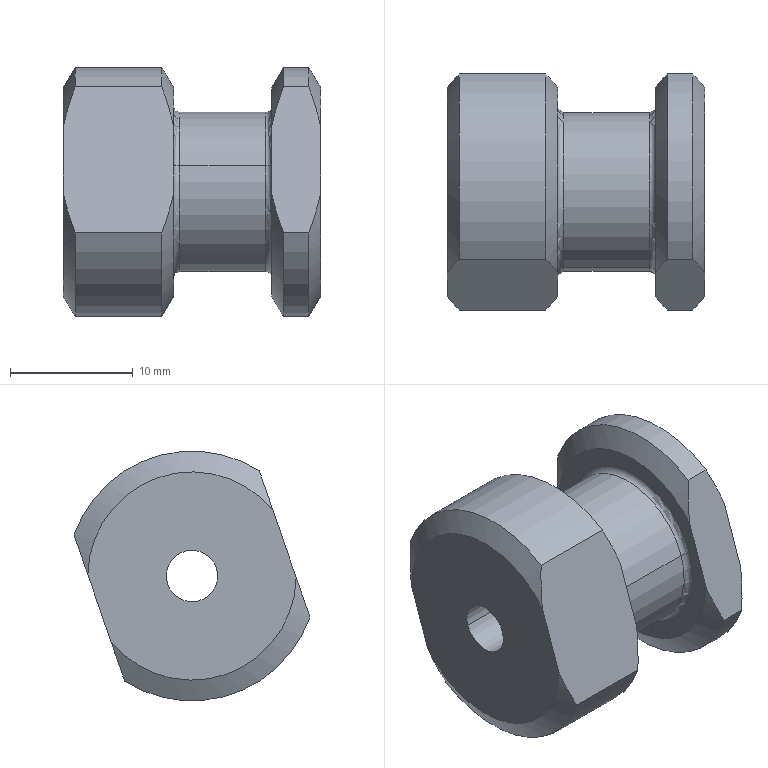Component | SolidWorks | 06-1111-1 | 1 solid | 28 faces | box 21 x 19.26 x 20.38 mm | volume 4401 mm3 | cylinder 8 | cone 8 | plane 8 | torus 4 | commonest cylinder face diameters 20.384 x4 4.2 x2 13 x2
build123d program:
from build123d import *

# Parameters (mm, degrees)
SKETCH2_OUTSIDE_W   = 29.518
SKETCH2_OUTSIDE_H   = 29.518
SKETCH2_OUTSIDE_W_2 = 16
SKETCH2_OUTSIDE_H_2 = 25
EXTRUDE1_DEPTH      = 22
M5_TAPPED_HOLE1_D   = 4.2


with BuildPart() as part:
    # Sketch1 → Revolve1 (revolve)
    with BuildSketch(Plane.XY, mode=Mode.PRIVATE) as revolve1_sk:
        with BuildLine():
            Line((0, 0), (0, 8.5))
            Line((0, 8.5), (0.9769, 10.192))
            Line((0.9769, 10.192), (3.023, 10.192))
            Line((3.023, 10.192), (4, 8.5))
            Line((4, 8.5), (4, 7))
            ThreePointArc((4, 7), (4.146, 6.646), (4.5, 6.5))
            Line((4.5, 6.5), (11.5, 6.5))
            ThreePointArc((11.5, 6.5), (11.854, 6.646), (12, 7))
            Line((12, 7), (12, 8.5))
            Line((12, 8.5), (12.977, 10.192))
            Line((12.977, 10.192), (20.023, 10.192))
            Line((20.023, 10.192), (21, 8.5))
            Line((21, 8.5), (21, 0))
            Line((21, 0), (0, 0))
        make_face()
    revolve(revolve1_sk.sketch.rotate(Axis((21, 0, 0), (-1, 0, 0)), 270), axis=Axis((21, 0, 0), (-1, 0, 0)))

    # Sketch2 outside → Extrude1 (cut)
    with BuildSketch(Plane(origin=(0, 0, 0), x_dir=(0, 0, -1), z_dir=(1, 0, 0))):
        Rectangle(SKETCH2_OUTSIDE_W, SKETCH2_OUTSIDE_H)
        Rectangle(SKETCH2_OUTSIDE_W_2, SKETCH2_OUTSIDE_H_2, mode=Mode.SUBTRACT)
    extrude(amount=EXTRUDE1_DEPTH, mode=Mode.SUBTRACT)

    # M5 Tapped Hole1 (through all)
    with Locations(Plane.ZY):
        with Locations((0, 0)):
            Hole(M5_TAPPED_HOLE1_D / 2)


solid = part.part

# Placed as in the assembly
solid = solid.moved(Location((-65, 24, -26), (-109.129, 0, 180)))
STEP:
#1=CARTESIAN_POINT('',(-3.386,0.8668,-0.9965));
#2=VERTEX_POINT('',#1);
#3=CARTESIAN_POINT('',(-3.386,1.023,-1.051));
#4=VERTEX_POINT('',#3);
#5=CARTESIAN_POINT('',(-3.386,0.9449,-1.024));
#6=DIRECTION('',(1.,0.,-0.));
#7=DIRECTION('',(0.,0.9448,-0.3277));
#8=AXIS2_PLACEMENT_3D('',#5,#6,#7);
#9=CIRCLE('',#8,0.08268);
#10=EDGE_CURVE('',#2,#4,#9,.T.);
#11=ORIENTED_EDGE('',*,*,#10,.F.);
#12=CARTESIAN_POINT('',(-2.559,0.8668,-0.9965));
#13=VERTEX_POINT('',#12);
#14=CARTESIAN_POINT('',(-2.559,0.8668,-0.9965));
#15=DIRECTION('',(1.,0.,-0.));
#16=VECTOR('',#15,39.37);
#17=LINE('',#14,#16);
#18=EDGE_CURVE('',#2,#13,#17,.T.);
#19=ORIENTED_EDGE('',*,*,#18,.T.);
#20=CARTESIAN_POINT('',(-2.559,1.023,-1.051));
#21=VERTEX_POINT('',#20);
#22=CARTESIAN_POINT('',(-2.559,0.9449,-1.024));
#23=DIRECTION('',(1.,0.,-0.));
#24=DIRECTION('',(0.,0.9448,-0.3277));
#25=AXIS2_PLACEMENT_3D('',#22,#23,#24);
#26=CIRCLE('',#25,0.08268);
#27=EDGE_CURVE('',#13,#21,#26,.T.);
#28=ORIENTED_EDGE('',*,*,#27,.T.);
#29=CARTESIAN_POINT('',(-2.559,1.023,-1.051));
#30=DIRECTION('',(1.,0.,-0.));
#31=VECTOR('',#30,39.37);
#32=LINE('',#29,#31);
#33=EDGE_CURVE('',#4,#21,#32,.T.);
#34=ORIENTED_EDGE('',*,*,#33,.F.);
#35=EDGE_LOOP('',(#11,#19,#28,#34));
#36=FACE_OUTER_BOUND('',#35,.T.);
#37=CARTESIAN_POINT('',(-2.559,0.9449,-1.024));
#38=DIRECTION('',(1.,0.,-0.));
#39=DIRECTION('',(0.,0.9448,-0.3277));
#40=AXIS2_PLACEMENT_3D('',#37,#38,#39);
#41=CYLINDRICAL_SURFACE('',#40,0.08268);
#42=ADVANCED_FACE('',(#36),#41,.F.);
#43=CARTESIAN_POINT('',(-2.717,0.6845,-0.9333));
#44=VERTEX_POINT('',#43);
#45=CARTESIAN_POINT('',(-2.717,1.205,-1.114));
#46=VERTEX_POINT('',#45);
#47=CARTESIAN_POINT('',(-2.717,0.9449,-1.024));
#48=DIRECTION('',(1.,0.,-0.));
#49=DIRECTION('',(0.,0.9448,-0.3277));
#50=AXIS2_PLACEMENT_3D('',#47,#48,#49);
#51=CIRCLE('',#50,0.2756);
#52=EDGE_CURVE('',#44,#46,#51,.T.);
#53=ORIENTED_EDGE('',*,*,#52,.F.);
#54=CARTESIAN_POINT('',(-2.736,0.7031,-0.9398));
#55=VERTEX_POINT('',#54);
#56=CARTESIAN_POINT('',(-2.736,0.6845,-0.9333));
#57=DIRECTION('',(0.,0.3277,0.9448));
#58=DIRECTION('',(0.,-0.9448,0.3277));
#59=AXIS2_PLACEMENT_3D('',#56,#57,#58);
#60=CIRCLE('',#59,0.01969);
#61=EDGE_CURVE('',#44,#55,#60,.T.);
#62=ORIENTED_EDGE('',*,*,#61,.T.);
#63=CARTESIAN_POINT('',(-2.736,1.187,-1.107));
#64=VERTEX_POINT('',#63);
#65=CARTESIAN_POINT('',(-2.736,0.9449,-1.024));
#66=DIRECTION('',(1.,0.,-0.));
#67=DIRECTION('',(0.,0.9448,-0.3277));
#68=AXIS2_PLACEMENT_3D('',#65,#66,#67);
#69=CIRCLE('',#68,0.2559);
#70=EDGE_CURVE('',#55,#64,#69,.T.);
#71=ORIENTED_EDGE('',*,*,#70,.T.);
#72=CARTESIAN_POINT('',(-2.736,1.205,-1.114));
#73=DIRECTION('',(-0.,-0.3277,-0.9448));
#74=DIRECTION('',(0.,0.9448,-0.3277));
#75=AXIS2_PLACEMENT_3D('',#72,#73,#74);
#76=CIRCLE('',#75,0.01969);
#77=EDGE_CURVE('',#46,#64,#76,.T.);
#78=ORIENTED_EDGE('',*,*,#77,.F.);
#79=EDGE_LOOP('',(#53,#62,#71,#78));
#80=FACE_OUTER_BOUND('',#79,.T.);
#81=CARTESIAN_POINT('',(-2.736,0.9449,-1.024));
#82=DIRECTION('',(1.,0.,-0.));
#83=DIRECTION('',(-0.,0.9448,-0.3277));
#84=AXIS2_PLACEMENT_3D('',#81,#82,#83);
#85=TOROIDAL_SURFACE('',#84,0.2756,0.01969);
#86=ADVANCED_FACE('',(#80),#85,.F.);
#87=CARTESIAN_POINT('',(-3.012,1.187,-1.107));
#88=VERTEX_POINT('',#87);
#89=CARTESIAN_POINT('',(-3.012,0.7031,-0.9398));
#90=VERTEX_POINT('',#89);
#91=CARTESIAN_POINT('',(-3.012,0.9449,-1.024));
#92=DIRECTION('',(1.,0.,-0.));
#93=DIRECTION('',(0.,0.9448,-0.3277));
#94=AXIS2_PLACEMENT_3D('',#91,#92,#93);
#95=CIRCLE('',#94,0.2559);
#96=EDGE_CURVE('',#88,#90,#95,.T.);
#97=ORIENTED_EDGE('',*,*,#96,.T.);
#98=CARTESIAN_POINT('',(-3.386,0.7031,-0.9398));
#99=DIRECTION('',(1.,0.,-0.));
#100=VECTOR('',#99,39.37);
#101=LINE('',#98,#100);
#102=EDGE_CURVE('',#90,#55,#101,.T.);
#103=ORIENTED_EDGE('',*,*,#102,.T.);
#104=CARTESIAN_POINT('',(-2.736,0.9449,-1.024));
#105=DIRECTION('',(1.,0.,-0.));
#106=DIRECTION('',(0.,0.9448,-0.3277));
#107=AXIS2_PLACEMENT_3D('',#104,#105,#106);
#108=CIRCLE('',#107,0.2559);
#109=EDGE_CURVE('',#64,#55,#108,.T.);
#110=ORIENTED_EDGE('',*,*,#109,.F.);
#111=CARTESIAN_POINT('',(-3.386,1.187,-1.107));
#112=DIRECTION('',(1.,0.,-0.));
#113=VECTOR('',#112,39.37);
#114=LINE('',#111,#113);
#115=EDGE_CURVE('',#88,#64,#114,.T.);
#116=ORIENTED_EDGE('',*,*,#115,.F.);
#117=EDGE_LOOP('',(#97,#103,#110,#116));
#118=FACE_OUTER_BOUND('',#117,.T.);
#119=CARTESIAN_POINT('',(-3.386,0.9449,-1.024));
#120=DIRECTION('',(1.,0.,-0.));
#121=DIRECTION('',(0.,0.9448,-0.3277));
#122=AXIS2_PLACEMENT_3D('',#119,#120,#121);
#123=CYLINDRICAL_SURFACE('',#122,0.2559);
#124=ADVANCED_FACE('',(#118),#123,.T.);
#125=CARTESIAN_POINT('',(-3.012,0.9449,-1.024));
#126=DIRECTION('',(1.,0.,-0.));
#127=DIRECTION('',(0.,0.9448,-0.3277));
#128=AXIS2_PLACEMENT_3D('',#125,#126,#127);
#129=CIRCLE('',#128,0.2559);
#130=EDGE_CURVE('',#90,#88,#129,.T.);
#131=ORIENTED_EDGE('',*,*,#130,.F.);
#132=CARTESIAN_POINT('',(-3.031,0.6845,-0.9333));
#133=VERTEX_POINT('',#132);
#134=CARTESIAN_POINT('',(-3.012,0.6845,-0.9333));
#135=DIRECTION('',(0.,0.3277,0.9448));
#136=DIRECTION('',(0.,-0.9448,0.3277));
#137=AXIS2_PLACEMENT_3D('',#134,#135,#136);
#138=CIRCLE('',#137,0.01969);
#139=EDGE_CURVE('',#90,#133,#138,.T.);
#140=ORIENTED_EDGE('',*,*,#139,.T.);
#141=CARTESIAN_POINT('',(-3.031,1.205,-1.114));
#142=VERTEX_POINT('',#141);
#143=CARTESIAN_POINT('',(-3.031,0.9449,-1.024));
#144=DIRECTION('',(1.,0.,-0.));
#145=DIRECTION('',(0.,0.9448,-0.3277));
#146=AXIS2_PLACEMENT_3D('',#143,#144,#145);
#147=CIRCLE('',#146,0.2756);
#148=EDGE_CURVE('',#133,#142,#147,.T.);
#149=ORIENTED_EDGE('',*,*,#148,.T.);
#150=CARTESIAN_POINT('',(-3.012,1.205,-1.114));
#151=DIRECTION('',(-0.,-0.3277,-0.9448));
#152=DIRECTION('',(0.,0.9448,-0.3277));
#153=AXIS2_PLACEMENT_3D('',#150,#151,#152);
#154=CIRCLE('',#153,0.01969);
#155=EDGE_CURVE('',#88,#142,#154,.T.);
#156=ORIENTED_EDGE('',*,*,#155,.F.);
#157=EDGE_LOOP('',(#131,#140,#149,#156));
#158=FACE_OUTER_BOUND('',#157,.T.);
#159=CARTESIAN_POINT('',(-3.012,0.9449,-1.024));
#160=DIRECTION('',(1.,0.,-0.));
#161=DIRECTION('',(-0.,0.9448,-0.3277));
#162=AXIS2_PLACEMENT_3D('',#159,#160,#161);
#163=TOROIDAL_SURFACE('',#162,0.2756,0.01969);
#164=ADVANCED_FACE('',(#158),#163,.F.);
#165=CARTESIAN_POINT('',(-3.347,1.324,-0.8919));
#166=VERTEX_POINT('',#165);
#167=CARTESIAN_POINT('',(-3.347,0.7288,-0.6855));
#168=VERTEX_POINT('',#167);
#169=CARTESIAN_POINT('',(-3.347,0.9449,-1.024));
#170=DIRECTION('',(1.,0.,-0.));
#171=DIRECTION('',(0.,0.9448,-0.3277));
#172=AXIS2_PLACEMENT_3D('',#169,#170,#171);
#173=CIRCLE('',#172,0.4013);
#174=EDGE_CURVE('',#166,#168,#173,.T.);
#175=ORIENTED_EDGE('',*,*,#174,.F.);
#176=CARTESIAN_POINT('',(-3.386,1.28,-1.02));
#177=VERTEX_POINT('',#176);
#178=CARTESIAN_POINT('',(-3.347,1.324,-0.8919));
#179=CARTESIAN_POINT('',(-3.355,1.317,-0.9128));
#180=CARTESIAN_POINT('',(-3.363,1.309,-0.9338));
#181=CARTESIAN_POINT('',(-3.376,1.295,-0.9765));
#182=CARTESIAN_POINT('',(-3.381,1.287,-0.9981));
#183=CARTESIAN_POINT('',(-3.386,1.28,-1.02));
#184=B_SPLINE_CURVE_WITH_KNOTS('',3,(#178,#179,#180,#181,#182,#183),.UNSPECIFIED.,.F.,.F.,(4,2,4),(0.01795,0.01974,0.02153),.UNSPECIFIED.);
#185=EDGE_CURVE('',#166,#177,#184,.T.);
#186=ORIENTED_EDGE('',*,*,#185,.T.);
#187=CARTESIAN_POINT('',(-3.386,0.6844,-0.8136));
#188=VERTEX_POINT('',#187);
#189=CARTESIAN_POINT('',(-3.386,0.9449,-1.024));
#190=DIRECTION('',(1.,0.,-0.));
#191=DIRECTION('',(0.,0.9448,-0.3277));
#192=AXIS2_PLACEMENT_3D('',#189,#190,#191);
#193=CIRCLE('',#192,0.3346);
#194=EDGE_CURVE('',#177,#188,#193,.T.);
#195=ORIENTED_EDGE('',*,*,#194,.T.);
#196=CARTESIAN_POINT('',(-3.386,0.6844,-0.8136));
#197=CARTESIAN_POINT('',(-3.377,0.6996,-0.7696));
#198=CARTESIAN_POINT('',(-3.363,0.7143,-0.7272));
#199=CARTESIAN_POINT('',(-3.347,0.7288,-0.6855));
#200=B_SPLINE_CURVE_WITH_KNOTS('',3,(#196,#197,#198,#199),.UNSPECIFIED.,.F.,.F.,(4,4),(0.02733,0.03094),.UNSPECIFIED.);
#201=EDGE_CURVE('',#188,#168,#200,.T.);
#202=ORIENTED_EDGE('',*,*,#201,.T.);
#203=EDGE_LOOP('',(#175,#186,#195,#202));
#204=FACE_OUTER_BOUND('',#203,.T.);
#205=CARTESIAN_POINT('',(-3.386,0.9449,-1.024));
#206=DIRECTION('',(1.,0.,-0.));
#207=DIRECTION('',(0.,0.9448,-0.3277));
#208=AXIS2_PLACEMENT_3D('',#205,#206,#207);
#209=CONICAL_SURFACE('',#208,0.3346,1.047);
#210=ADVANCED_FACE('',(#204),#209,.T.);
#211=CARTESIAN_POINT('',(-3.347,0.5658,-1.155));
#212=VERTEX_POINT('',#211);
#213=CARTESIAN_POINT('',(-3.347,1.161,-1.362));
#214=VERTEX_POINT('',#213);
#215=CARTESIAN_POINT('',(-3.347,0.9449,-1.024));
#216=DIRECTION('',(1.,0.,-0.));
#217=DIRECTION('',(0.,0.9448,-0.3277));
#218=AXIS2_PLACEMENT_3D('',#215,#216,#217);
#219=CIRCLE('',#218,0.4013);
#220=EDGE_CURVE('',#212,#214,#219,.T.);
#221=ORIENTED_EDGE('',*,*,#220,.T.);
#222=CARTESIAN_POINT('',(-3.07,1.161,-1.362));
#223=VERTEX_POINT('',#222);
#224=CARTESIAN_POINT('',(-3.386,1.161,-1.362));
#225=DIRECTION('',(1.,0.,-0.));
#226=VECTOR('',#225,39.37);
#227=LINE('',#224,#226);
#228=EDGE_CURVE('',#214,#223,#227,.T.);
#229=ORIENTED_EDGE('',*,*,#228,.T.);
#230=CARTESIAN_POINT('',(-3.07,0.5658,-1.155));
#231=VERTEX_POINT('',#230);
#232=CARTESIAN_POINT('',(-3.07,0.9449,-1.024));
#233=DIRECTION('',(1.,0.,-0.));
#234=DIRECTION('',(0.,0.9448,-0.3277));
#235=AXIS2_PLACEMENT_3D('',#232,#233,#234);
#236=CIRCLE('',#235,0.4013);
#237=EDGE_CURVE('',#231,#223,#236,.T.);
#238=ORIENTED_EDGE('',*,*,#237,.F.);
#239=CARTESIAN_POINT('',(-3.386,0.5658,-1.155));
#240=DIRECTION('',(-1.,-0.,0.));
#241=VECTOR('',#240,39.37);
#242=LINE('',#239,#241);
#243=EDGE_CURVE('',#231,#212,#242,.T.);
#244=ORIENTED_EDGE('',*,*,#243,.T.);
#245=EDGE_LOOP('',(#221,#229,#238,#244));
#246=FACE_OUTER_BOUND('',#245,.T.);
#247=CARTESIAN_POINT('',(-3.386,0.9449,-1.024));
#248=DIRECTION('',(1.,0.,-0.));
#249=DIRECTION('',(0.,0.9448,-0.3277));
#250=AXIS2_PLACEMENT_3D('',#247,#248,#249);
#251=CYLINDRICAL_SURFACE('',#250,0.4013);
#252=ADVANCED_FACE('',(#246),#251,.T.);
#253=ORIENTED_EDGE('',*,*,#237,.T.);
#254=CARTESIAN_POINT('',(-3.031,1.205,-1.234));
#255=VERTEX_POINT('',#254);
#256=CARTESIAN_POINT('',(-3.07,1.161,-1.362));
#257=CARTESIAN_POINT('',(-3.062,1.168,-1.341));
#258=CARTESIAN_POINT('',(-3.055,1.176,-1.32));
#259=CARTESIAN_POINT('',(-3.042,1.19,-1.277));
#260=CARTESIAN_POINT('',(-3.036,1.198,-1.256));
#261=CARTESIAN_POINT('',(-3.031,1.205,-1.234));
#262=B_SPLINE_CURVE_WITH_KNOTS('',3,(#256,#257,#258,#259,#260,#261),.UNSPECIFIED.,.F.,.F.,(4,2,4),(0.01795,0.01974,0.02153),.UNSPECIFIED.);
#263=EDGE_CURVE('',#223,#255,#262,.T.);
#264=ORIENTED_EDGE('',*,*,#263,.T.);
#265=CARTESIAN_POINT('',(-3.031,0.6103,-1.027));
#266=VERTEX_POINT('',#265);
#267=CARTESIAN_POINT('',(-3.031,0.9449,-1.024));
#268=DIRECTION('',(1.,0.,-0.));
#269=DIRECTION('',(0.,0.9448,-0.3277));
#270=AXIS2_PLACEMENT_3D('',#267,#268,#269);
#271=CIRCLE('',#270,0.3346);
#272=EDGE_CURVE('',#266,#255,#271,.T.);
#273=ORIENTED_EDGE('',*,*,#272,.F.);
#274=CARTESIAN_POINT('',(-3.031,0.6103,-1.027));
#275=CARTESIAN_POINT('',(-3.041,0.595,-1.071));
#276=CARTESIAN_POINT('',(-3.054,0.5803,-1.114));
#277=CARTESIAN_POINT('',(-3.07,0.5658,-1.155));
#278=B_SPLINE_CURVE_WITH_KNOTS('',3,(#274,#275,#276,#277),.UNSPECIFIED.,.F.,.F.,(4,4),(0.02733,0.03094),.UNSPECIFIED.);
#279=EDGE_CURVE('',#266,#231,#278,.T.);
#280=ORIENTED_EDGE('',*,*,#279,.T.);
#281=EDGE_LOOP('',(#253,#264,#273,#280));
#282=FACE_OUTER_BOUND('',#281,.T.);
#283=CARTESIAN_POINT('',(-3.07,0.9449,-1.024));
#284=DIRECTION('',(-1.,-0.,0.));
#285=DIRECTION('',(0.,-0.9448,0.3277));
#286=AXIS2_PLACEMENT_3D('',#283,#284,#285);
#287=CONICAL_SURFACE('',#286,0.4013,1.047);
#288=ADVANCED_FACE('',(#282),#287,.T.);
#289=CARTESIAN_POINT('',(-2.678,1.324,-0.8919));
#290=VERTEX_POINT('',#289);
#291=CARTESIAN_POINT('',(-2.678,0.7288,-0.6855));
#292=VERTEX_POINT('',#291);
#293=CARTESIAN_POINT('',(-2.678,0.9449,-1.024));
#294=DIRECTION('',(1.,0.,-0.));
#295=DIRECTION('',(0.,0.9448,-0.3277));
#296=AXIS2_PLACEMENT_3D('',#293,#294,#295);
#297=CIRCLE('',#296,0.4013);
#298=EDGE_CURVE('',#290,#292,#297,.T.);
#299=ORIENTED_EDGE('',*,*,#298,.F.);
#300=CARTESIAN_POINT('',(-2.717,1.28,-1.02));
#301=VERTEX_POINT('',#300);
#302=CARTESIAN_POINT('',(-2.678,1.324,-0.8919));
#303=CARTESIAN_POINT('',(-2.686,1.317,-0.9128));
#304=CARTESIAN_POINT('',(-2.693,1.309,-0.9338));
#305=CARTESIAN_POINT('',(-2.706,1.295,-0.9765));
#306=CARTESIAN_POINT('',(-2.712,1.287,-0.9981));
#307=CARTESIAN_POINT('',(-2.717,1.28,-1.02));
#308=B_SPLINE_CURVE_WITH_KNOTS('',3,(#302,#303,#304,#305,#306,#307),.UNSPECIFIED.,.F.,.F.,(4,2,4),(0.01795,0.01974,0.02153),.UNSPECIFIED.);
#309=EDGE_CURVE('',#290,#301,#308,.T.);
#310=ORIENTED_EDGE('',*,*,#309,.T.);
#311=CARTESIAN_POINT('',(-2.717,0.6844,-0.8136));
#312=VERTEX_POINT('',#311);
#313=CARTESIAN_POINT('',(-2.717,0.9449,-1.024));
#314=DIRECTION('',(1.,0.,-0.));
#315=DIRECTION('',(0.,0.9448,-0.3277));
#316=AXIS2_PLACEMENT_3D('',#313,#314,#315);
#317=CIRCLE('',#316,0.3346);
#318=EDGE_CURVE('',#301,#312,#317,.T.);
#319=ORIENTED_EDGE('',*,*,#318,.T.);
#320=CARTESIAN_POINT('',(-2.717,0.6844,-0.8136));
#321=CARTESIAN_POINT('',(-2.707,0.6996,-0.7696));
#322=CARTESIAN_POINT('',(-2.694,0.7143,-0.7272));
#323=CARTESIAN_POINT('',(-2.678,0.7288,-0.6855));
#324=B_SPLINE_CURVE_WITH_KNOTS('',3,(#320,#321,#322,#323),.UNSPECIFIED.,.F.,.F.,(4,4),(0.02733,0.03094),.UNSPECIFIED.);
#325=EDGE_CURVE('',#312,#292,#324,.T.);
#326=ORIENTED_EDGE('',*,*,#325,.T.);
#327=EDGE_LOOP('',(#299,#310,#319,#326));
#328=FACE_OUTER_BOUND('',#327,.T.);
#329=CARTESIAN_POINT('',(-2.717,0.9449,-1.024));
#330=DIRECTION('',(1.,0.,-0.));
#331=DIRECTION('',(0.,0.9448,-0.3277));
#332=AXIS2_PLACEMENT_3D('',#329,#330,#331);
#333=CONICAL_SURFACE('',#332,0.3346,1.047);
#334=ADVANCED_FACE('',(#328),#333,.T.);
#335=CARTESIAN_POINT('',(-2.678,0.5658,-1.155));
#336=VERTEX_POINT('',#335);
#337=CARTESIAN_POINT('',(-2.678,1.161,-1.362));
#338=VERTEX_POINT('',#337);
#339=CARTESIAN_POINT('',(-2.678,0.9449,-1.024));
#340=DIRECTION('',(1.,0.,-0.));
#341=DIRECTION('',(0.,0.9448,-0.3277));
#342=AXIS2_PLACEMENT_3D('',#339,#340,#341);
#343=CIRCLE('',#342,0.4013);
#344=EDGE_CURVE('',#336,#338,#343,.T.);
#345=ORIENTED_EDGE('',*,*,#344,.T.);
#346=CARTESIAN_POINT('',(-2.598,1.161,-1.362));
#347=VERTEX_POINT('',#346);
#348=CARTESIAN_POINT('',(-3.386,1.161,-1.362));
#349=DIRECTION('',(1.,0.,-0.));
#350=VECTOR('',#349,39.37);
#351=LINE('',#348,#350);
#352=EDGE_CURVE('',#338,#347,#351,.T.);
#353=ORIENTED_EDGE('',*,*,#352,.T.);
#354=CARTESIAN_POINT('',(-2.598,0.5658,-1.155));
#355=VERTEX_POINT('',#354);
#356=CARTESIAN_POINT('',(-2.598,0.9449,-1.024));
#357=DIRECTION('',(1.,0.,-0.));
#358=DIRECTION('',(0.,0.9448,-0.3277));
#359=AXIS2_PLACEMENT_3D('',#356,#357,#358);
#360=CIRCLE('',#359,0.4013);
#361=EDGE_CURVE('',#355,#347,#360,.T.);
#362=ORIENTED_EDGE('',*,*,#361,.F.);
#363=CARTESIAN_POINT('',(-3.386,0.5658,-1.155));
#364=DIRECTION('',(-1.,-0.,0.));
#365=VECTOR('',#364,39.37);
#366=LINE('',#363,#365);
#367=EDGE_CURVE('',#355,#336,#366,.T.);
#368=ORIENTED_EDGE('',*,*,#367,.T.);
#369=EDGE_LOOP('',(#345,#353,#362,#368));
#370=FACE_OUTER_BOUND('',#369,.T.);
#371=CARTESIAN_POINT('',(-3.386,0.9449,-1.024));
#372=DIRECTION('',(1.,0.,-0.));
#373=DIRECTION('',(0.,0.9448,-0.3277));
#374=AXIS2_PLACEMENT_3D('',#371,#372,#373);
#375=CYLINDRICAL_SURFACE('',#374,0.4013);
#376=ADVANCED_FACE('',(#370),#375,.T.);
#377=ORIENTED_EDGE('',*,*,#361,.T.);
#378=CARTESIAN_POINT('',(-2.559,1.205,-1.234));
#379=VERTEX_POINT('',#378);
#380=CARTESIAN_POINT('',(-2.598,1.161,-1.362));
#381=CARTESIAN_POINT('',(-2.59,1.168,-1.341));
#382=CARTESIAN_POINT('',(-2.582,1.176,-1.32));
#383=CARTESIAN_POINT('',(-2.569,1.19,-1.277));
#384=CARTESIAN_POINT('',(-2.564,1.198,-1.256));
#385=CARTESIAN_POINT('',(-2.559,1.205,-1.234));
#386=B_SPLINE_CURVE_WITH_KNOTS('',3,(#380,#381,#382,#383,#384,#385),.UNSPECIFIED.,.F.,.F.,(4,2,4),(0.01795,0.01974,0.02153),.UNSPECIFIED.);
#387=EDGE_CURVE('',#347,#379,#386,.T.);
#388=ORIENTED_EDGE('',*,*,#387,.T.);
#389=CARTESIAN_POINT('',(-2.559,0.6103,-1.027));
#390=VERTEX_POINT('',#389);
#391=CARTESIAN_POINT('',(-2.559,0.9449,-1.024));
#392=DIRECTION('',(1.,0.,-0.));
#393=DIRECTION('',(0.,0.9448,-0.3277));
#394=AXIS2_PLACEMENT_3D('',#391,#392,#393);
#395=CIRCLE('',#394,0.3346);
#396=EDGE_CURVE('',#390,#379,#395,.T.);
#397=ORIENTED_EDGE('',*,*,#396,.F.);
#398=CARTESIAN_POINT('',(-2.559,0.6103,-1.027));
#399=CARTESIAN_POINT('',(-2.568,0.595,-1.071));
#400=CARTESIAN_POINT('',(-2.582,0.5803,-1.114));
#401=CARTESIAN_POINT('',(-2.598,0.5658,-1.155));
#402=B_SPLINE_CURVE_WITH_KNOTS('',3,(#398,#399,#400,#401),.UNSPECIFIED.,.F.,.F.,(4,4),(0.02733,0.03094),.UNSPECIFIED.);
#403=EDGE_CURVE('',#390,#355,#402,.T.);
#404=ORIENTED_EDGE('',*,*,#403,.T.);
#405=EDGE_LOOP('',(#377,#388,#397,#404));
#406=FACE_OUTER_BOUND('',#405,.T.);
#407=CARTESIAN_POINT('',(-2.598,0.9449,-1.024));
#408=DIRECTION('',(-1.,-0.,0.));
#409=DIRECTION('',(0.,-0.9448,0.3277));
#410=AXIS2_PLACEMENT_3D('',#407,#408,#409);
#411=CONICAL_SURFACE('',#410,0.4013,1.047);
#412=ADVANCED_FACE('',(#406),#411,.T.);
#413=CARTESIAN_POINT('',(-3.386,0.9449,-1.024));
#414=DIRECTION('',(1.,0.,-0.));
#415=DIRECTION('',(0.,0.9448,-0.3277));
#416=AXIS2_PLACEMENT_3D('',#413,#414,#415);
#417=CIRCLE('',#416,0.08268);
#418=EDGE_CURVE('',#4,#2,#417,.T.);
#419=ORIENTED_EDGE('',*,*,#418,.T.);
#420=ORIENTED_EDGE('',*,*,#10,.T.);
#421=EDGE_LOOP('',(#419,#420));
#422=FACE_BOUND('',#421,.T.);
#423=ORIENTED_EDGE('',*,*,#194,.F.);
#424=CARTESIAN_POINT('',(-3.386,1.205,-1.234));
#425=VERTEX_POINT('',#424);
#426=CARTESIAN_POINT('',(-3.386,1.352,-0.8107));
#427=DIRECTION('',(-0.,-0.3277,-0.9448));
#428=VECTOR('',#427,39.37);
#429=LINE('',#426,#428);
#430=EDGE_CURVE('',#177,#425,#429,.T.);
#431=ORIENTED_EDGE('',*,*,#430,.T.);
#432=CARTESIAN_POINT('',(-3.386,0.6103,-1.027));
#433=VERTEX_POINT('',#432);
#434=CARTESIAN_POINT('',(-3.386,0.9449,-1.024));
#435=DIRECTION('',(1.,0.,-0.));
#436=DIRECTION('',(0.,0.9448,-0.3277));
#437=AXIS2_PLACEMENT_3D('',#434,#435,#436);
#438=CIRCLE('',#437,0.3346);
#439=EDGE_CURVE('',#433,#425,#438,.T.);
#440=ORIENTED_EDGE('',*,*,#439,.F.);
#441=CARTESIAN_POINT('',(-3.386,0.757,-0.6042));
#442=DIRECTION('',(0.,0.3277,0.9448));
#443=VECTOR('',#442,39.37);
#444=LINE('',#441,#443);
#445=EDGE_CURVE('',#433,#188,#444,.T.);
#446=ORIENTED_EDGE('',*,*,#445,.T.);
#447=EDGE_LOOP('',(#423,#431,#440,#446));
#448=FACE_OUTER_BOUND('',#447,.T.);
#449=CARTESIAN_POINT('',(-3.386,1.055,-0.7075));
#450=DIRECTION('',(1.,0.,-0.));
#451=DIRECTION('',(-0.,0.9448,-0.3277));
#452=AXIS2_PLACEMENT_3D('',#449,#450,#451);
#453=PLANE('',#452);
#454=ADVANCED_FACE('',(#422,#448),#453,.F.);
#455=ORIENTED_EDGE('',*,*,#439,.T.);
#456=CARTESIAN_POINT('',(-3.386,1.205,-1.234));
#457=CARTESIAN_POINT('',(-3.377,1.19,-1.278));
#458=CARTESIAN_POINT('',(-3.363,1.175,-1.32));
#459=CARTESIAN_POINT('',(-3.347,1.161,-1.362));
#460=B_SPLINE_CURVE_WITH_KNOTS('',3,(#456,#457,#458,#459),.UNSPECIFIED.,.F.,.F.,(4,4),(0.02733,0.03094),.UNSPECIFIED.);
#461=EDGE_CURVE('',#425,#214,#460,.T.);
#462=ORIENTED_EDGE('',*,*,#461,.T.);
#463=ORIENTED_EDGE('',*,*,#220,.F.);
#464=CARTESIAN_POINT('',(-3.347,0.5658,-1.155));
#465=CARTESIAN_POINT('',(-3.355,0.5731,-1.134));
#466=CARTESIAN_POINT('',(-3.363,0.5804,-1.113));
#467=CARTESIAN_POINT('',(-3.376,0.5952,-1.071));
#468=CARTESIAN_POINT('',(-3.381,0.6027,-1.049));
#469=CARTESIAN_POINT('',(-3.386,0.6103,-1.027));
#470=B_SPLINE_CURVE_WITH_KNOTS('',3,(#464,#465,#466,#467,#468,#469),.UNSPECIFIED.,.F.,.F.,(4,2,4),(0.01795,0.01974,0.02153),.UNSPECIFIED.);
#471=EDGE_CURVE('',#212,#433,#470,.T.);
#472=ORIENTED_EDGE('',*,*,#471,.T.);
#473=EDGE_LOOP('',(#455,#462,#463,#472));
#474=FACE_OUTER_BOUND('',#473,.T.);
#475=CARTESIAN_POINT('',(-3.386,0.9449,-1.024));
#476=DIRECTION('',(1.,0.,-0.));
#477=DIRECTION('',(0.,0.9448,-0.3277));
#478=AXIS2_PLACEMENT_3D('',#475,#476,#477);
#479=CONICAL_SURFACE('',#478,0.3346,1.047);
#480=ADVANCED_FACE('',(#474),#479,.T.);
#481=CARTESIAN_POINT('',(-3.07,1.324,-0.8919));
#482=VERTEX_POINT('',#481);
#483=CARTESIAN_POINT('',(-3.07,0.7288,-0.6855));
#484=VERTEX_POINT('',#483);
#485=CARTESIAN_POINT('',(-3.07,0.9449,-1.024));
#486=DIRECTION('',(1.,0.,-0.));
#487=DIRECTION('',(0.,0.9448,-0.3277));
#488=AXIS2_PLACEMENT_3D('',#485,#486,#487);
#489=CIRCLE('',#488,0.4013);
#490=EDGE_CURVE('',#482,#484,#489,.T.);
#491=ORIENTED_EDGE('',*,*,#490,.F.);
#492=CARTESIAN_POINT('',(-3.386,1.324,-0.8919));
#493=DIRECTION('',(-1.,-0.,0.));
#494=VECTOR('',#493,39.37);
#495=LINE('',#492,#494);
#496=EDGE_CURVE('',#482,#166,#495,.T.);
#497=ORIENTED_EDGE('',*,*,#496,.T.);
#498=ORIENTED_EDGE('',*,*,#174,.T.);
#499=CARTESIAN_POINT('',(-3.386,0.7288,-0.6855));
#500=DIRECTION('',(1.,0.,-0.));
#501=VECTOR('',#500,39.37);
#502=LINE('',#499,#501);
#503=EDGE_CURVE('',#168,#484,#502,.T.);
#504=ORIENTED_EDGE('',*,*,#503,.T.);
#505=EDGE_LOOP('',(#491,#497,#498,#504));
#506=FACE_OUTER_BOUND('',#505,.T.);
#507=CARTESIAN_POINT('',(-3.386,0.9449,-1.024));
#508=DIRECTION('',(1.,0.,-0.));
#509=DIRECTION('',(0.,0.9448,-0.3277));
#510=AXIS2_PLACEMENT_3D('',#507,#508,#509);
#511=CYLINDRICAL_SURFACE('',#510,0.4013);
#512=ADVANCED_FACE('',(#506),#511,.T.);
#513=CARTESIAN_POINT('',(-3.031,1.28,-1.02));
#514=VERTEX_POINT('',#513);
#515=CARTESIAN_POINT('',(-3.031,0.6844,-0.8136));
#516=VERTEX_POINT('',#515);
#517=CARTESIAN_POINT('',(-3.031,0.9449,-1.024));
#518=DIRECTION('',(1.,0.,-0.));
#519=DIRECTION('',(0.,0.9448,-0.3277));
#520=AXIS2_PLACEMENT_3D('',#517,#518,#519);
#521=CIRCLE('',#520,0.3346);
#522=EDGE_CURVE('',#514,#516,#521,.T.);
#523=ORIENTED_EDGE('',*,*,#522,.F.);
#524=CARTESIAN_POINT('',(-3.031,1.28,-1.02));
#525=CARTESIAN_POINT('',(-3.041,1.295,-0.9761));
#526=CARTESIAN_POINT('',(-3.054,1.309,-0.9336));
#527=CARTESIAN_POINT('',(-3.07,1.324,-0.8919));
#528=B_SPLINE_CURVE_WITH_KNOTS('',3,(#524,#525,#526,#527),.UNSPECIFIED.,.F.,.F.,(4,4),(0.02733,0.03094),.UNSPECIFIED.);
#529=EDGE_CURVE('',#514,#482,#528,.T.);
#530=ORIENTED_EDGE('',*,*,#529,.T.);
#531=ORIENTED_EDGE('',*,*,#490,.T.);
#532=CARTESIAN_POINT('',(-3.07,0.7288,-0.6855));
#533=CARTESIAN_POINT('',(-3.062,0.7216,-0.7064));
#534=CARTESIAN_POINT('',(-3.055,0.7143,-0.7274));
#535=CARTESIAN_POINT('',(-3.042,0.6995,-0.77));
#536=CARTESIAN_POINT('',(-3.036,0.6919,-0.7917));
#537=CARTESIAN_POINT('',(-3.031,0.6844,-0.8136));
#538=B_SPLINE_CURVE_WITH_KNOTS('',3,(#532,#533,#534,#535,#536,#537),.UNSPECIFIED.,.F.,.F.,(4,2,4),(0.01795,0.01974,0.02153),.UNSPECIFIED.);
#539=EDGE_CURVE('',#484,#516,#538,.T.);
#540=ORIENTED_EDGE('',*,*,#539,.T.);
#541=EDGE_LOOP('',(#523,#530,#531,#540));
#542=FACE_OUTER_BOUND('',#541,.T.);
#543=CARTESIAN_POINT('',(-3.07,0.9449,-1.024));
#544=DIRECTION('',(-1.,-0.,0.));
#545=DIRECTION('',(0.,-0.9448,0.3277));
#546=AXIS2_PLACEMENT_3D('',#543,#544,#545);
#547=CONICAL_SURFACE('',#546,0.4013,1.047);
#548=ADVANCED_FACE('',(#542),#547,.T.);
#549=CARTESIAN_POINT('',(-3.031,0.9449,-1.024));
#550=DIRECTION('',(1.,0.,-0.));
#551=DIRECTION('',(0.,0.9448,-0.3277));
#552=AXIS2_PLACEMENT_3D('',#549,#550,#551);
#553=CIRCLE('',#552,0.2756);
#554=EDGE_CURVE('',#142,#133,#553,.T.);
#555=ORIENTED_EDGE('',*,*,#554,.F.);
#556=ORIENTED_EDGE('',*,*,#148,.F.);
#557=EDGE_LOOP('',(#555,#556));
#558=FACE_BOUND('',#557,.T.);
#559=ORIENTED_EDGE('',*,*,#272,.T.);
#560=CARTESIAN_POINT('',(-3.031,1.333,-0.8665));
#561=DIRECTION('',(0.,0.3277,0.9448));
#562=VECTOR('',#561,39.37);
#563=LINE('',#560,#562);
#564=EDGE_CURVE('',#255,#514,#563,.T.);
#565=ORIENTED_EDGE('',*,*,#564,.T.);
#566=ORIENTED_EDGE('',*,*,#522,.T.);
#567=CARTESIAN_POINT('',(-3.031,0.7376,-0.66));
#568=DIRECTION('',(-0.,-0.3277,-0.9448));
#569=VECTOR('',#568,39.37);
#570=LINE('',#567,#569);
#571=EDGE_CURVE('',#516,#266,#570,.T.);
#572=ORIENTED_EDGE('',*,*,#571,.T.);
#573=EDGE_LOOP('',(#559,#565,#566,#572));
#574=FACE_OUTER_BOUND('',#573,.T.);
#575=CARTESIAN_POINT('',(-3.031,1.035,-0.7632));
#576=DIRECTION('',(-1.,-0.,0.));
#577=DIRECTION('',(0.,-0.9448,0.3277));
#578=AXIS2_PLACEMENT_3D('',#575,#576,#577);
#579=PLANE('',#578);
#580=ADVANCED_FACE('',(#558,#574),#579,.F.);
#581=ORIENTED_EDGE('',*,*,#139,.F.);
#582=ORIENTED_EDGE('',*,*,#96,.F.);
#583=ORIENTED_EDGE('',*,*,#155,.T.);
#584=ORIENTED_EDGE('',*,*,#554,.T.);
#585=EDGE_LOOP('',(#581,#582,#583,#584));
#586=FACE_OUTER_BOUND('',#585,.T.);
#587=CARTESIAN_POINT('',(-3.012,0.9449,-1.024));
#588=DIRECTION('',(1.,0.,-0.));
#589=DIRECTION('',(-0.,0.9448,-0.3277));
#590=AXIS2_PLACEMENT_3D('',#587,#588,#589);
#591=TOROIDAL_SURFACE('',#590,0.2756,0.01969);
#592=ADVANCED_FACE('',(#586),#591,.F.);
#593=ORIENTED_EDGE('',*,*,#102,.F.);
#594=ORIENTED_EDGE('',*,*,#130,.T.);
#595=ORIENTED_EDGE('',*,*,#115,.T.);
#596=ORIENTED_EDGE('',*,*,#70,.F.);
#597=EDGE_LOOP('',(#593,#594,#595,#596));
#598=FACE_OUTER_BOUND('',#597,.T.);
#599=CARTESIAN_POINT('',(-3.386,0.9449,-1.024));
#600=DIRECTION('',(1.,0.,-0.));
#601=DIRECTION('',(0.,0.9448,-0.3277));
#602=AXIS2_PLACEMENT_3D('',#599,#600,#601);
#603=CYLINDRICAL_SURFACE('',#602,0.2559);
#604=ADVANCED_FACE('',(#598),#603,.T.);
#605=ORIENTED_EDGE('',*,*,#61,.F.);
#606=CARTESIAN_POINT('',(-2.717,0.9449,-1.024));
#607=DIRECTION('',(1.,0.,-0.));
#608=DIRECTION('',(0.,0.9448,-0.3277));
#609=AXIS2_PLACEMENT_3D('',#606,#607,#608);
#610=CIRCLE('',#609,0.2756);
#611=EDGE_CURVE('',#46,#44,#610,.T.);
#612=ORIENTED_EDGE('',*,*,#611,.F.);
#613=ORIENTED_EDGE('',*,*,#77,.T.);
#614=ORIENTED_EDGE('',*,*,#109,.T.);
#615=EDGE_LOOP('',(#605,#612,#613,#614));
#616=FACE_OUTER_BOUND('',#615,.T.);
#617=CARTESIAN_POINT('',(-2.736,0.9449,-1.024));
#618=DIRECTION('',(1.,0.,-0.));
#619=DIRECTION('',(-0.,0.9448,-0.3277));
#620=AXIS2_PLACEMENT_3D('',#617,#618,#619);
#621=TOROIDAL_SURFACE('',#620,0.2756,0.01969);
#622=ADVANCED_FACE('',(#616),#621,.F.);
#623=ORIENTED_EDGE('',*,*,#318,.F.);
#624=CARTESIAN_POINT('',(-2.717,1.205,-1.234));
#625=VERTEX_POINT('',#624);
#626=CARTESIAN_POINT('',(-2.717,1.352,-0.8107));
#627=DIRECTION('',(-0.,-0.3277,-0.9448));
#628=VECTOR('',#627,39.37);
#629=LINE('',#626,#628);
#630=EDGE_CURVE('',#301,#625,#629,.T.);
#631=ORIENTED_EDGE('',*,*,#630,.T.);
#632=CARTESIAN_POINT('',(-2.717,0.6103,-1.027));
#633=VERTEX_POINT('',#632);
#634=CARTESIAN_POINT('',(-2.717,0.9449,-1.024));
#635=DIRECTION('',(1.,0.,-0.));
#636=DIRECTION('',(0.,0.9448,-0.3277));
#637=AXIS2_PLACEMENT_3D('',#634,#635,#636);
#638=CIRCLE('',#637,0.3346);
#639=EDGE_CURVE('',#633,#625,#638,.T.);
#640=ORIENTED_EDGE('',*,*,#639,.F.);
#641=CARTESIAN_POINT('',(-2.717,0.757,-0.6042));
#642=DIRECTION('',(0.,0.3277,0.9448));
#643=VECTOR('',#642,39.37);
#644=LINE('',#641,#643);
#645=EDGE_CURVE('',#633,#312,#644,.T.);
#646=ORIENTED_EDGE('',*,*,#645,.T.);
#647=EDGE_LOOP('',(#623,#631,#640,#646));
#648=FACE_OUTER_BOUND('',#647,.T.);
#649=ORIENTED_EDGE('',*,*,#611,.T.);
#650=ORIENTED_EDGE('',*,*,#52,.T.);
#651=EDGE_LOOP('',(#649,#650));
#652=FACE_BOUND('',#651,.T.);
#653=CARTESIAN_POINT('',(-2.717,1.055,-0.7075));
#654=DIRECTION('',(1.,0.,-0.));
#655=DIRECTION('',(-0.,0.9448,-0.3277));
#656=AXIS2_PLACEMENT_3D('',#653,#654,#655);
#657=PLANE('',#656);
#658=ADVANCED_FACE('',(#648,#652),#657,.F.);
#659=ORIENTED_EDGE('',*,*,#639,.T.);
#660=CARTESIAN_POINT('',(-2.717,1.205,-1.234));
#661=CARTESIAN_POINT('',(-2.707,1.19,-1.278));
#662=CARTESIAN_POINT('',(-2.694,1.175,-1.32));
#663=CARTESIAN_POINT('',(-2.678,1.161,-1.362));
#664=B_SPLINE_CURVE_WITH_KNOTS('',3,(#660,#661,#662,#663),.UNSPECIFIED.,.F.,.F.,(4,4),(0.02733,0.03094),.UNSPECIFIED.);
#665=EDGE_CURVE('',#625,#338,#664,.T.);
#666=ORIENTED_EDGE('',*,*,#665,.T.);
#667=ORIENTED_EDGE('',*,*,#344,.F.);
#668=CARTESIAN_POINT('',(-2.678,0.5658,-1.155));
#669=CARTESIAN_POINT('',(-2.686,0.5731,-1.134));
#670=CARTESIAN_POINT('',(-2.693,0.5804,-1.113));
#671=CARTESIAN_POINT('',(-2.706,0.5952,-1.071));
#672=CARTESIAN_POINT('',(-2.712,0.6027,-1.049));
#673=CARTESIAN_POINT('',(-2.717,0.6103,-1.027));
#674=B_SPLINE_CURVE_WITH_KNOTS('',3,(#668,#669,#670,#671,#672,#673),.UNSPECIFIED.,.F.,.F.,(4,2,4),(0.01795,0.01974,0.02153),.UNSPECIFIED.);
#675=EDGE_CURVE('',#336,#633,#674,.T.);
#676=ORIENTED_EDGE('',*,*,#675,.T.);
#677=EDGE_LOOP('',(#659,#666,#667,#676));
#678=FACE_OUTER_BOUND('',#677,.T.);
#679=CARTESIAN_POINT('',(-2.717,0.9449,-1.024));
#680=DIRECTION('',(1.,0.,-0.));
#681=DIRECTION('',(0.,0.9448,-0.3277));
#682=AXIS2_PLACEMENT_3D('',#679,#680,#681);
#683=CONICAL_SURFACE('',#682,0.3346,1.047);
#684=ADVANCED_FACE('',(#678),#683,.T.);
#685=CARTESIAN_POINT('',(-2.598,1.324,-0.8919));
#686=VERTEX_POINT('',#685);
#687=CARTESIAN_POINT('',(-2.598,0.7288,-0.6855));
#688=VERTEX_POINT('',#687);
#689=CARTESIAN_POINT('',(-2.598,0.9449,-1.024));
#690=DIRECTION('',(1.,0.,-0.));
#691=DIRECTION('',(0.,0.9448,-0.3277));
#692=AXIS2_PLACEMENT_3D('',#689,#690,#691);
#693=CIRCLE('',#692,0.4013);
#694=EDGE_CURVE('',#686,#688,#693,.T.);
#695=ORIENTED_EDGE('',*,*,#694,.F.);
#696=CARTESIAN_POINT('',(-3.386,1.324,-0.8919));
#697=DIRECTION('',(-1.,-0.,0.));
#698=VECTOR('',#697,39.37);
#699=LINE('',#696,#698);
#700=EDGE_CURVE('',#686,#290,#699,.T.);
#701=ORIENTED_EDGE('',*,*,#700,.T.);
#702=ORIENTED_EDGE('',*,*,#298,.T.);
#703=CARTESIAN_POINT('',(-3.386,0.7288,-0.6855));
#704=DIRECTION('',(1.,0.,-0.));
#705=VECTOR('',#704,39.37);
#706=LINE('',#703,#705);
#707=EDGE_CURVE('',#292,#688,#706,.T.);
#708=ORIENTED_EDGE('',*,*,#707,.T.);
#709=EDGE_LOOP('',(#695,#701,#702,#708));
#710=FACE_OUTER_BOUND('',#709,.T.);
#711=CARTESIAN_POINT('',(-3.386,0.9449,-1.024));
#712=DIRECTION('',(1.,0.,-0.));
#713=DIRECTION('',(0.,0.9448,-0.3277));
#714=AXIS2_PLACEMENT_3D('',#711,#712,#713);
#715=CYLINDRICAL_SURFACE('',#714,0.4013);
#716=ADVANCED_FACE('',(#710),#715,.T.);
#717=CARTESIAN_POINT('',(-2.559,1.28,-1.02));
#718=VERTEX_POINT('',#717);
#719=CARTESIAN_POINT('',(-2.559,0.6844,-0.8136));
#720=VERTEX_POINT('',#719);
#721=CARTESIAN_POINT('',(-2.559,0.9449,-1.024));
#722=DIRECTION('',(1.,0.,-0.));
#723=DIRECTION('',(0.,0.9448,-0.3277));
#724=AXIS2_PLACEMENT_3D('',#721,#722,#723);
#725=CIRCLE('',#724,0.3346);
#726=EDGE_CURVE('',#718,#720,#725,.T.);
#727=ORIENTED_EDGE('',*,*,#726,.F.);
#728=CARTESIAN_POINT('',(-2.559,1.28,-1.02));
#729=CARTESIAN_POINT('',(-2.568,1.295,-0.9761));
#730=CARTESIAN_POINT('',(-2.582,1.309,-0.9336));
#731=CARTESIAN_POINT('',(-2.598,1.324,-0.8919));
#732=B_SPLINE_CURVE_WITH_KNOTS('',3,(#728,#729,#730,#731),.UNSPECIFIED.,.F.,.F.,(4,4),(0.02733,0.03094),.UNSPECIFIED.);
#733=EDGE_CURVE('',#718,#686,#732,.T.);
#734=ORIENTED_EDGE('',*,*,#733,.T.);
#735=ORIENTED_EDGE('',*,*,#694,.T.);
#736=CARTESIAN_POINT('',(-2.598,0.7288,-0.6855));
#737=CARTESIAN_POINT('',(-2.59,0.7216,-0.7064));
#738=CARTESIAN_POINT('',(-2.582,0.7143,-0.7274));
#739=CARTESIAN_POINT('',(-2.569,0.6995,-0.77));
#740=CARTESIAN_POINT('',(-2.564,0.6919,-0.7917));
#741=CARTESIAN_POINT('',(-2.559,0.6844,-0.8136));
#742=B_SPLINE_CURVE_WITH_KNOTS('',3,(#736,#737,#738,#739,#740,#741),.UNSPECIFIED.,.F.,.F.,(4,2,4),(0.01795,0.01974,0.02153),.UNSPECIFIED.);
#743=EDGE_CURVE('',#688,#720,#742,.T.);
#744=ORIENTED_EDGE('',*,*,#743,.T.);
#745=EDGE_LOOP('',(#727,#734,#735,#744));
#746=FACE_OUTER_BOUND('',#745,.T.);
#747=CARTESIAN_POINT('',(-2.598,0.9449,-1.024));
#748=DIRECTION('',(-1.,-0.,0.));
#749=DIRECTION('',(0.,-0.9448,0.3277));
#750=AXIS2_PLACEMENT_3D('',#747,#748,#749);
#751=CONICAL_SURFACE('',#750,0.4013,1.047);
#752=ADVANCED_FACE('',(#746),#751,.T.);
#753=CARTESIAN_POINT('',(-2.559,0.9449,-1.024));
#754=DIRECTION('',(1.,0.,-0.));
#755=DIRECTION('',(0.,0.9448,-0.3277));
#756=AXIS2_PLACEMENT_3D('',#753,#754,#755);
#757=CIRCLE('',#756,0.08268);
#758=EDGE_CURVE('',#21,#13,#757,.T.);
#759=ORIENTED_EDGE('',*,*,#758,.F.);
#760=ORIENTED_EDGE('',*,*,#27,.F.);
#761=EDGE_LOOP('',(#759,#760));
#762=FACE_BOUND('',#761,.T.);
#763=ORIENTED_EDGE('',*,*,#396,.T.);
#764=CARTESIAN_POINT('',(-2.559,1.242,-1.127));
#765=DIRECTION('',(0.,0.3277,0.9448));
#766=VECTOR('',#765,39.37);
#767=LINE('',#764,#766);
#768=EDGE_CURVE('',#379,#718,#767,.T.);
#769=ORIENTED_EDGE('',*,*,#768,.T.);
#770=ORIENTED_EDGE('',*,*,#726,.T.);
#771=CARTESIAN_POINT('',(-2.559,0.6473,-0.9204));
#772=DIRECTION('',(-0.,-0.3277,-0.9448));
#773=VECTOR('',#772,39.37);
#774=LINE('',#771,#773);
#775=EDGE_CURVE('',#720,#390,#774,.T.);
#776=ORIENTED_EDGE('',*,*,#775,.T.);
#777=EDGE_LOOP('',(#763,#769,#770,#776));
#778=FACE_OUTER_BOUND('',#777,.T.);
#779=CARTESIAN_POINT('',(-2.559,0.9449,-1.024));
#780=DIRECTION('',(-1.,-0.,0.));
#781=DIRECTION('',(0.,-0.9448,0.3277));
#782=AXIS2_PLACEMENT_3D('',#779,#780,#781);
#783=PLANE('',#782);
#784=ADVANCED_FACE('',(#762,#778),#783,.F.);
#785=ORIENTED_EDGE('',*,*,#707,.F.);
#786=ORIENTED_EDGE('',*,*,#325,.F.);
#787=ORIENTED_EDGE('',*,*,#645,.F.);
#788=ORIENTED_EDGE('',*,*,#675,.F.);
#789=ORIENTED_EDGE('',*,*,#367,.F.);
#790=ORIENTED_EDGE('',*,*,#403,.F.);
#791=ORIENTED_EDGE('',*,*,#775,.F.);
#792=ORIENTED_EDGE('',*,*,#743,.F.);
#793=EDGE_LOOP('',(#785,#786,#787,#788,#789,#790,#791,#792));
#794=FACE_OUTER_BOUND('',#793,.T.);
#795=CARTESIAN_POINT('',(-3.425,0.8086,-0.4555));
#796=DIRECTION('',(-0.,0.9448,-0.3277));
#797=DIRECTION('',(-0.,-0.3277,-0.9448));
#798=AXIS2_PLACEMENT_3D('',#795,#796,#797);
#799=PLANE('',#798);
#800=ADVANCED_FACE('',(#794),#799,.F.);
#801=ORIENTED_EDGE('',*,*,#352,.F.);
#802=ORIENTED_EDGE('',*,*,#665,.F.);
#803=ORIENTED_EDGE('',*,*,#630,.F.);
#804=ORIENTED_EDGE('',*,*,#309,.F.);
#805=ORIENTED_EDGE('',*,*,#700,.F.);
#806=ORIENTED_EDGE('',*,*,#733,.F.);
#807=ORIENTED_EDGE('',*,*,#768,.F.);
#808=ORIENTED_EDGE('',*,*,#387,.F.);
#809=EDGE_LOOP('',(#801,#802,#803,#804,#805,#806,#807,#808));
#810=FACE_OUTER_BOUND('',#809,.T.);
#811=CARTESIAN_POINT('',(-3.425,1.404,-0.6619));
#812=DIRECTION('',(0.,-0.9448,0.3277));
#813=DIRECTION('',(0.,0.3277,0.9448));
#814=AXIS2_PLACEMENT_3D('',#811,#812,#813);
#815=PLANE('',#814);
#816=ADVANCED_FACE('',(#810),#815,.F.);
#817=ORIENTED_EDGE('',*,*,#471,.F.);
#818=ORIENTED_EDGE('',*,*,#243,.F.);
#819=ORIENTED_EDGE('',*,*,#279,.F.);
#820=ORIENTED_EDGE('',*,*,#571,.F.);
#821=ORIENTED_EDGE('',*,*,#539,.F.);
#822=ORIENTED_EDGE('',*,*,#503,.F.);
#823=ORIENTED_EDGE('',*,*,#201,.F.);
#824=ORIENTED_EDGE('',*,*,#445,.F.);
#825=EDGE_LOOP('',(#817,#818,#819,#820,#821,#822,#823,#824));
#826=FACE_OUTER_BOUND('',#825,.T.);
#827=CARTESIAN_POINT('',(-3.425,0.8086,-0.4555));
#828=DIRECTION('',(-0.,0.9448,-0.3277));
#829=DIRECTION('',(-0.,-0.3277,-0.9448));
#830=AXIS2_PLACEMENT_3D('',#827,#828,#829);
#831=PLANE('',#830);
#832=ADVANCED_FACE('',(#826),#831,.F.);
#833=ORIENTED_EDGE('',*,*,#185,.F.);
#834=ORIENTED_EDGE('',*,*,#496,.F.);
#835=ORIENTED_EDGE('',*,*,#529,.F.);
#836=ORIENTED_EDGE('',*,*,#564,.F.);
#837=ORIENTED_EDGE('',*,*,#263,.F.);
#838=ORIENTED_EDGE('',*,*,#228,.F.);
#839=ORIENTED_EDGE('',*,*,#461,.F.);
#840=ORIENTED_EDGE('',*,*,#430,.F.);
#841=EDGE_LOOP('',(#833,#834,#835,#836,#837,#838,#839,#840));
#842=FACE_OUTER_BOUND('',#841,.T.);
#843=CARTESIAN_POINT('',(-3.425,1.404,-0.6619));
#844=DIRECTION('',(0.,-0.9448,0.3277));
#845=DIRECTION('',(0.,0.3277,0.9448));
#846=AXIS2_PLACEMENT_3D('',#843,#844,#845);
#847=PLANE('',#846);
#848=ADVANCED_FACE('',(#842),#847,.F.);
#849=ORIENTED_EDGE('',*,*,#18,.F.);
#850=ORIENTED_EDGE('',*,*,#418,.F.);
#851=ORIENTED_EDGE('',*,*,#33,.T.);
#852=ORIENTED_EDGE('',*,*,#758,.T.);
#853=EDGE_LOOP('',(#849,#850,#851,#852));
#854=FACE_OUTER_BOUND('',#853,.T.);
#855=CARTESIAN_POINT('',(-2.559,0.9449,-1.024));
#856=DIRECTION('',(1.,0.,-0.));
#857=DIRECTION('',(0.,0.9448,-0.3277));
#858=AXIS2_PLACEMENT_3D('',#855,#856,#857);
#859=CYLINDRICAL_SURFACE('',#858,0.08268);
#860=ADVANCED_FACE('',(#854),#859,.F.);
#861=CLOSED_SHELL('',(#42,#86,#124,#164,#210,#252,#288,#334,#376,#412,#454,#480,#512,#548,#580,#592,#604,#622,#658,#684,#716,#752,#784,#800,#816,#832,#848,#860));
#862=MANIFOLD_SOLID_BREP('',#861);
#863=CARTESIAN_POINT('',(0.,0.,0.));
#864=DIRECTION('',(0.,0.,1.));
#865=DIRECTION('',(1.,0.,0.));
#866=AXIS2_PLACEMENT_3D('',#863,#864,#865);
#867=(LENGTH_UNIT()NAMED_UNIT(*)SI_UNIT($,.METRE.));
#868=LENGTH_MEASURE_WITH_UNIT(LENGTH_MEASURE(0.0254),#867);
#869=DIMENSIONAL_EXPONENTS(1.,0.,0.,0.,0.,0.,0.);
#870=(CONVERSION_BASED_UNIT('',#868)LENGTH_UNIT()NAMED_UNIT(#869));
#871=UNCERTAINTY_MEASURE_WITH_UNIT(LENGTH_MEASURE(0.00001),#870,'','');
#872=(NAMED_UNIT(*)PLANE_ANGLE_UNIT()SI_UNIT($,.RADIAN.));
#873=(NAMED_UNIT(*)SI_UNIT($,.STERADIAN.)SOLID_ANGLE_UNIT());
#874=(GEOMETRIC_REPRESENTATION_CONTEXT(3)GLOBAL_UNCERTAINTY_ASSIGNED_CONTEXT((#871))GLOBAL_UNIT_ASSIGNED_CONTEXT((#870,#872,#873))REPRESENTATION_CONTEXT('',''));
#875=ADVANCED_BREP_SHAPE_REPRESENTATION('',(#862,#866),#874);
#876=COLOUR_RGB('',0.7922,0.8196,0.9333);
#877=FILL_AREA_STYLE_COLOUR('',#876);
#878=FILL_AREA_STYLE('',(#877));
#879=SURFACE_STYLE_FILL_AREA(#878);
#880=SURFACE_SIDE_STYLE('',(#879));
#881=SURFACE_STYLE_USAGE(.BOTH.,#880);
#882=PRESENTATION_STYLE_ASSIGNMENT((#881));
#883=STYLED_ITEM('',(#882),#862);
#884=PRESENTATION_LAYER_ASSIGNMENT('','',(#883));
#885=(LENGTH_UNIT()NAMED_UNIT(*)SI_UNIT($,.METRE.));
#886=LENGTH_MEASURE_WITH_UNIT(LENGTH_MEASURE(0.0254),#885);
#887=DIMENSIONAL_EXPONENTS(1.,0.,0.,0.,0.,0.,0.);
#888=(CONVERSION_BASED_UNIT('',#886)LENGTH_UNIT()NAMED_UNIT(#887));
#889=UNCERTAINTY_MEASURE_WITH_UNIT(LENGTH_MEASURE(0.00001),#888,'','');
#890=(NAMED_UNIT(*)PLANE_ANGLE_UNIT()SI_UNIT($,.RADIAN.));
#891=(NAMED_UNIT(*)SI_UNIT($,.STERADIAN.)SOLID_ANGLE_UNIT());
#892=(GEOMETRIC_REPRESENTATION_CONTEXT(3)GLOBAL_UNCERTAINTY_ASSIGNED_CONTEXT((#889))GLOBAL_UNIT_ASSIGNED_CONTEXT((#888,#890,#891))REPRESENTATION_CONTEXT('',''));
#893=MECHANICAL_DESIGN_GEOMETRIC_PRESENTATION_REPRESENTATION('',(#883),#892);